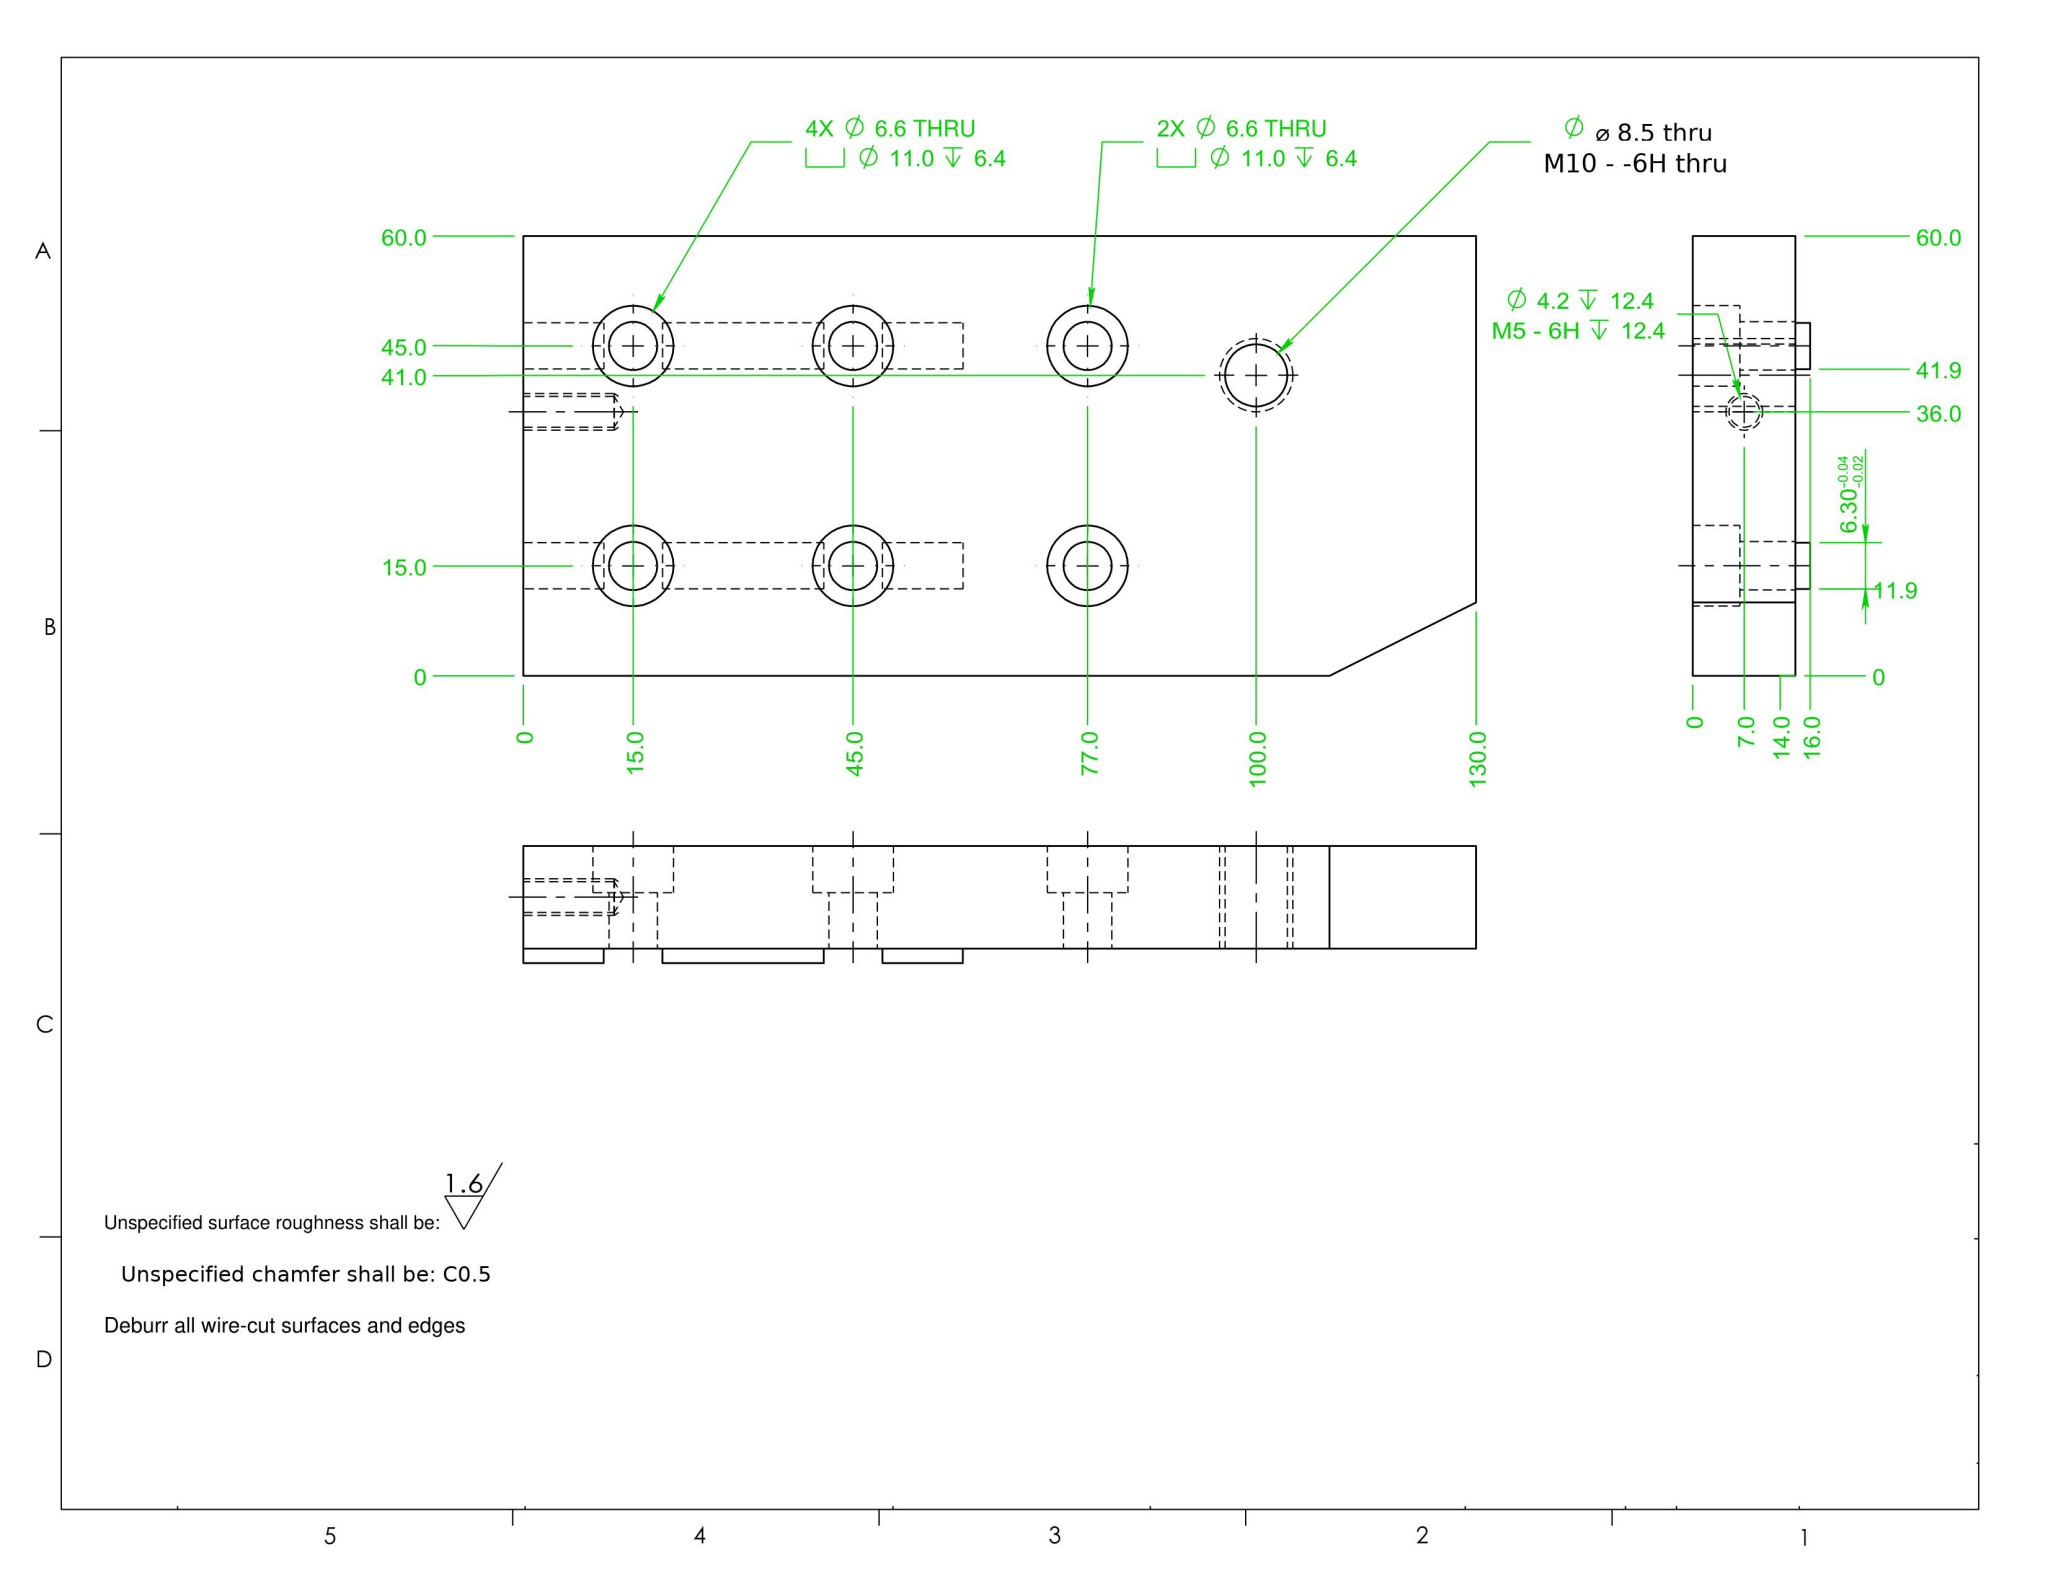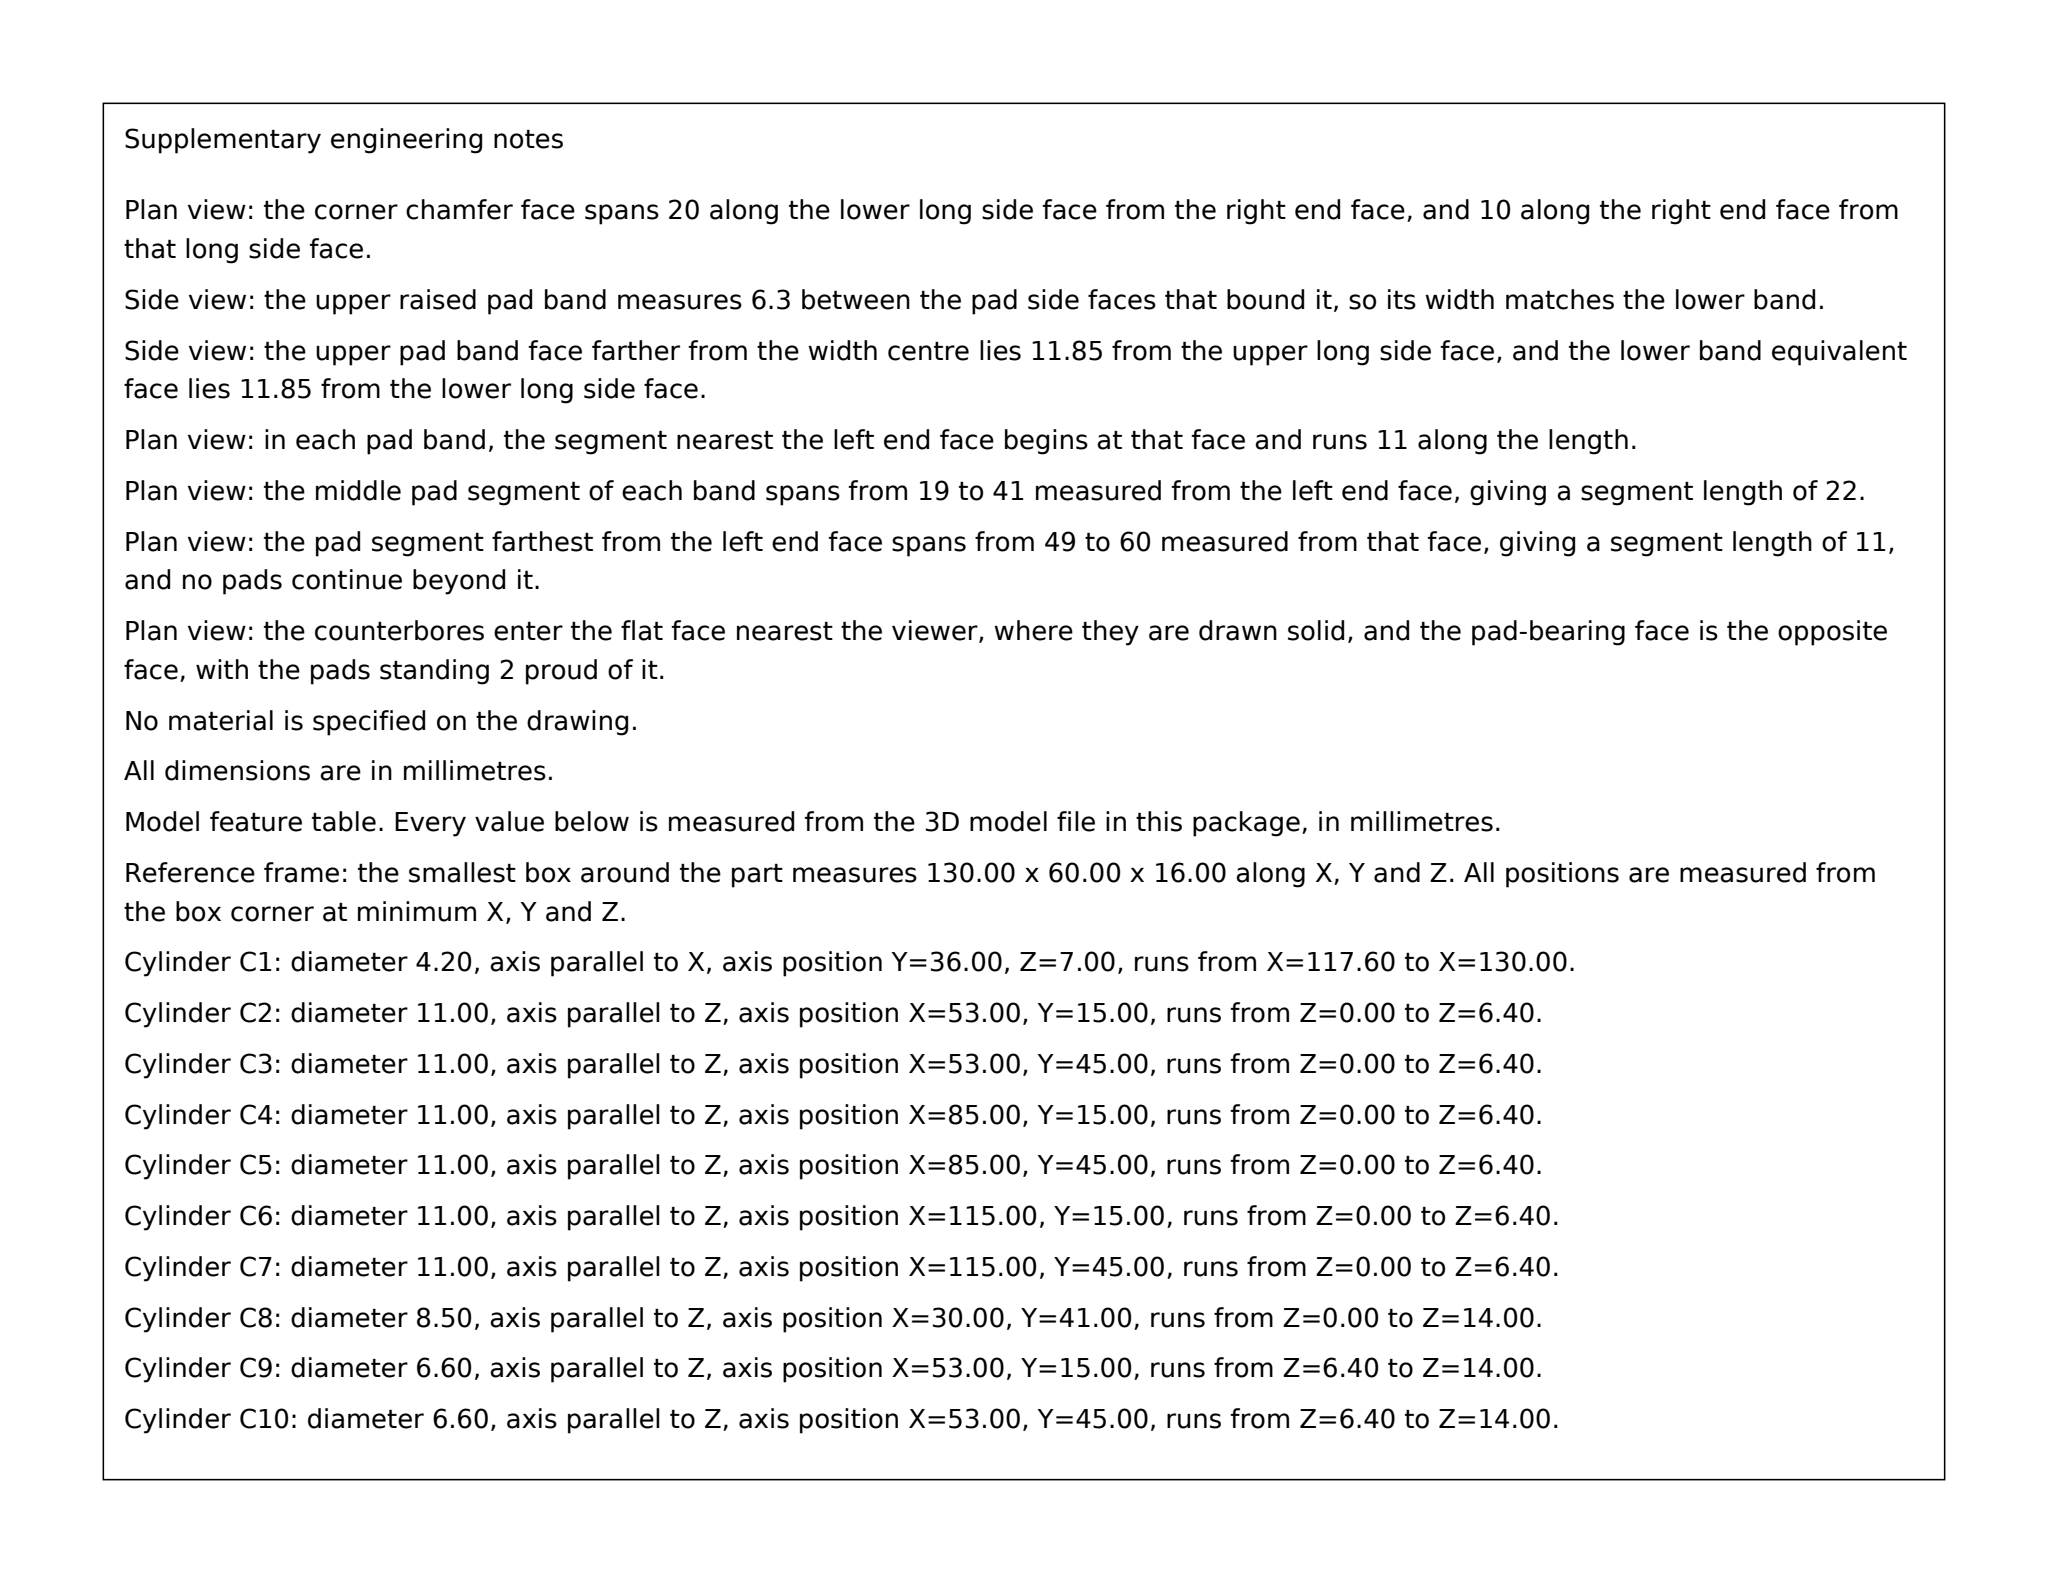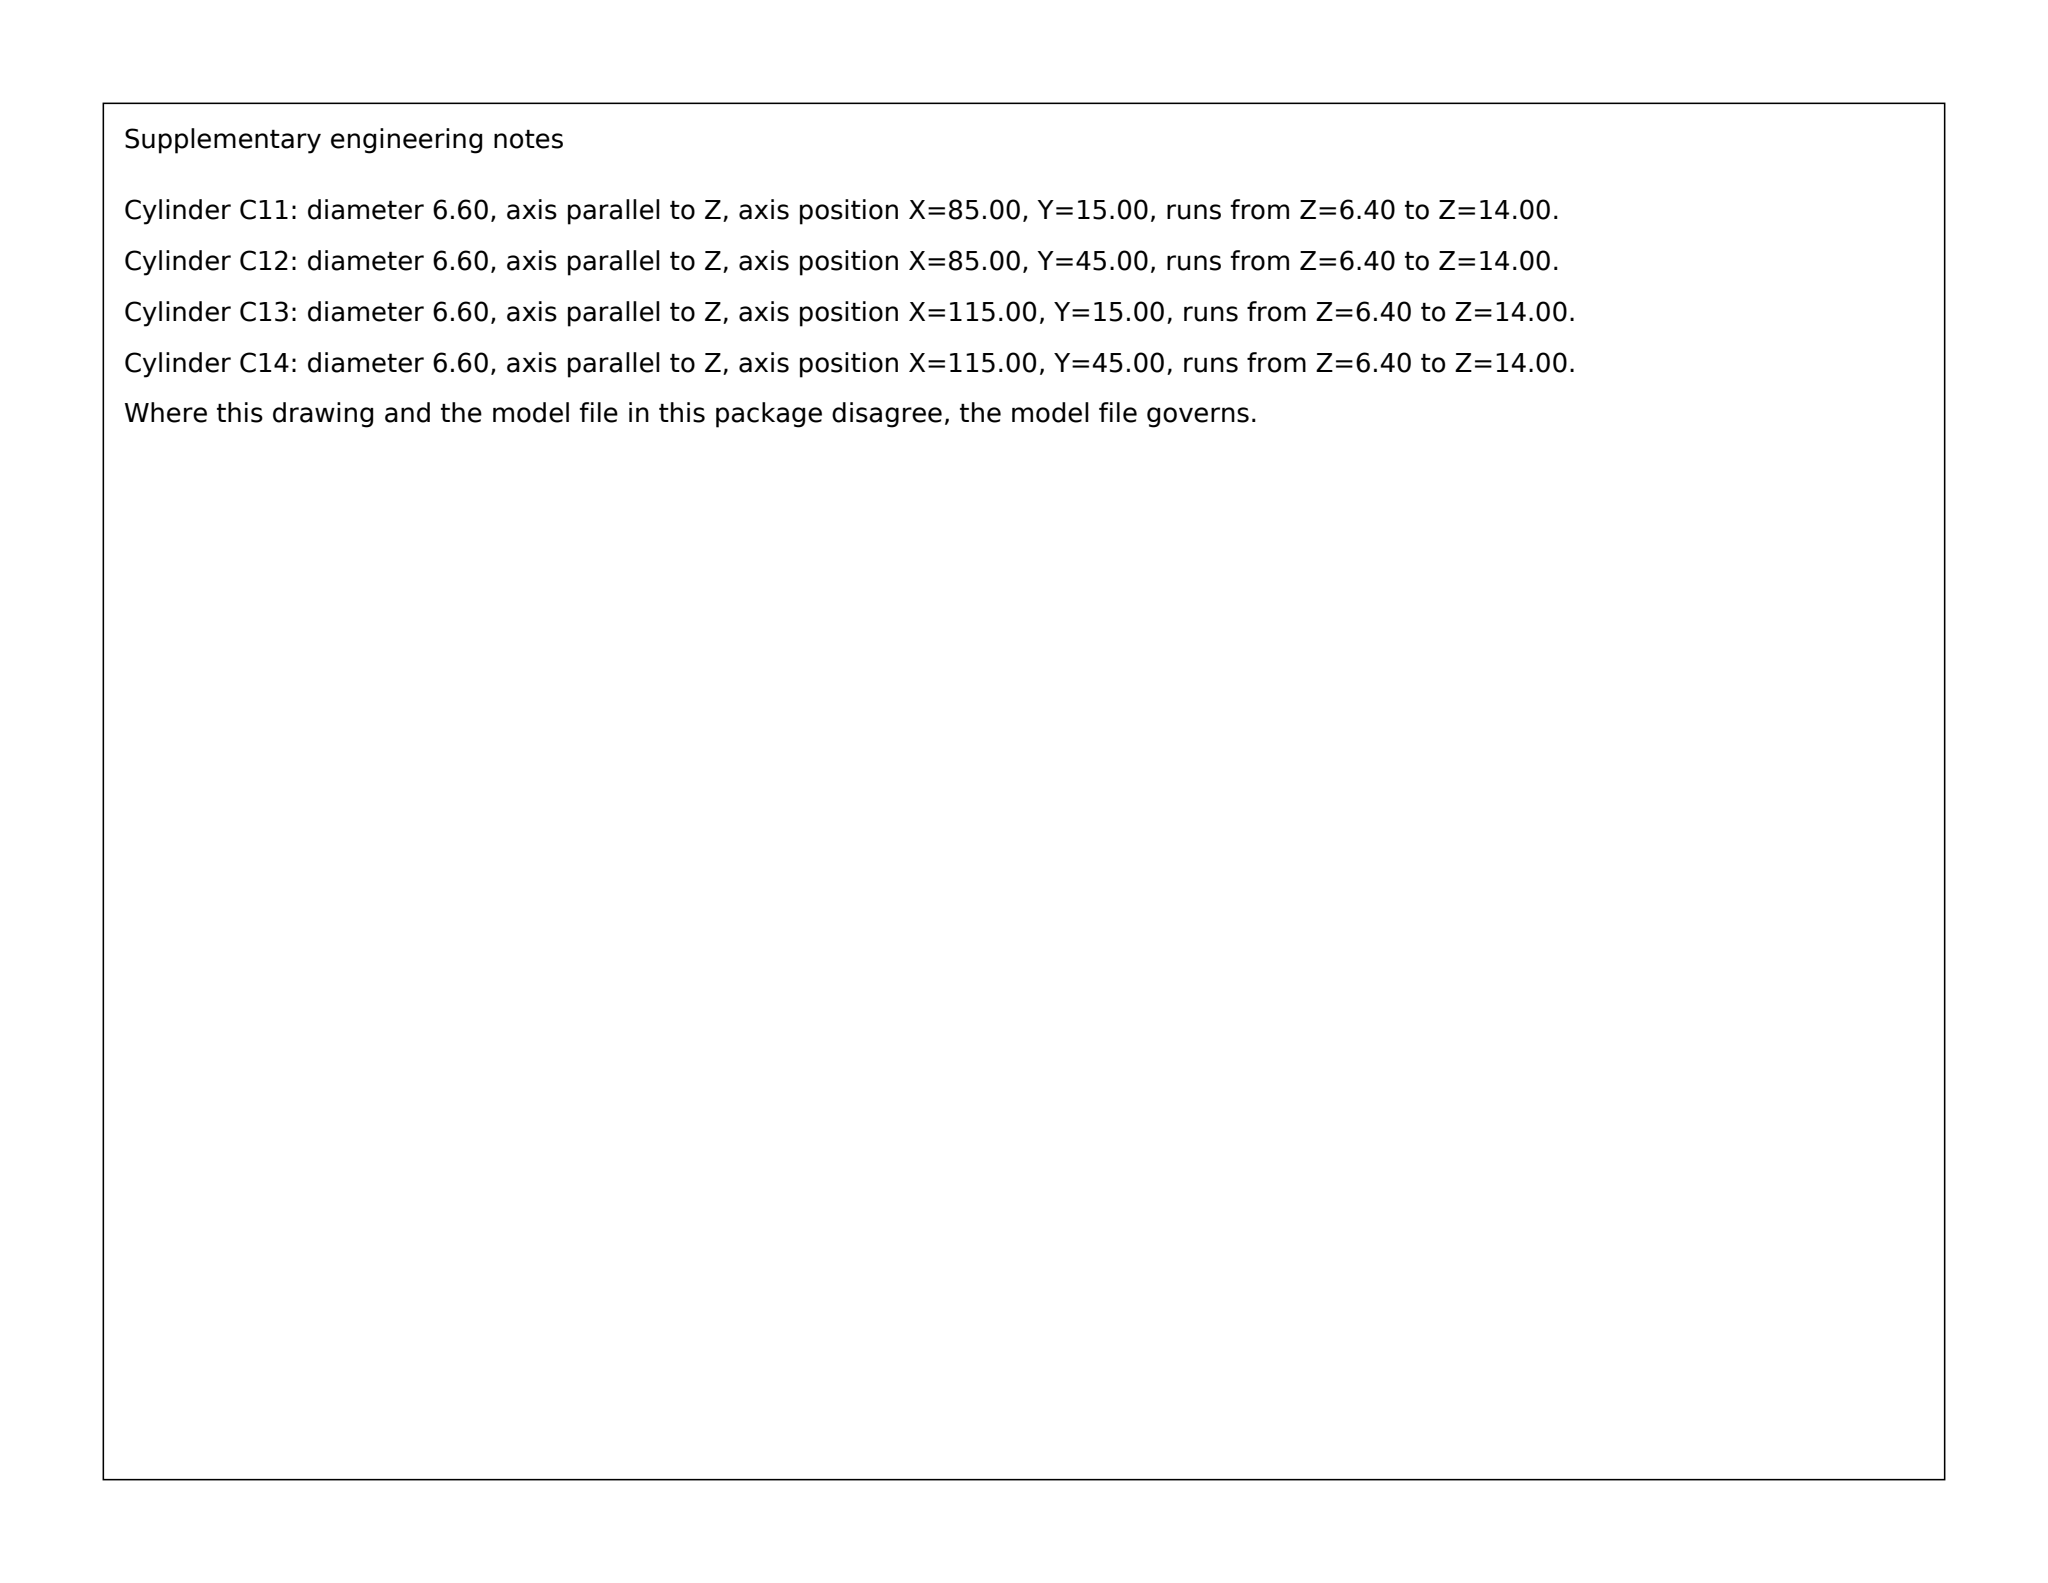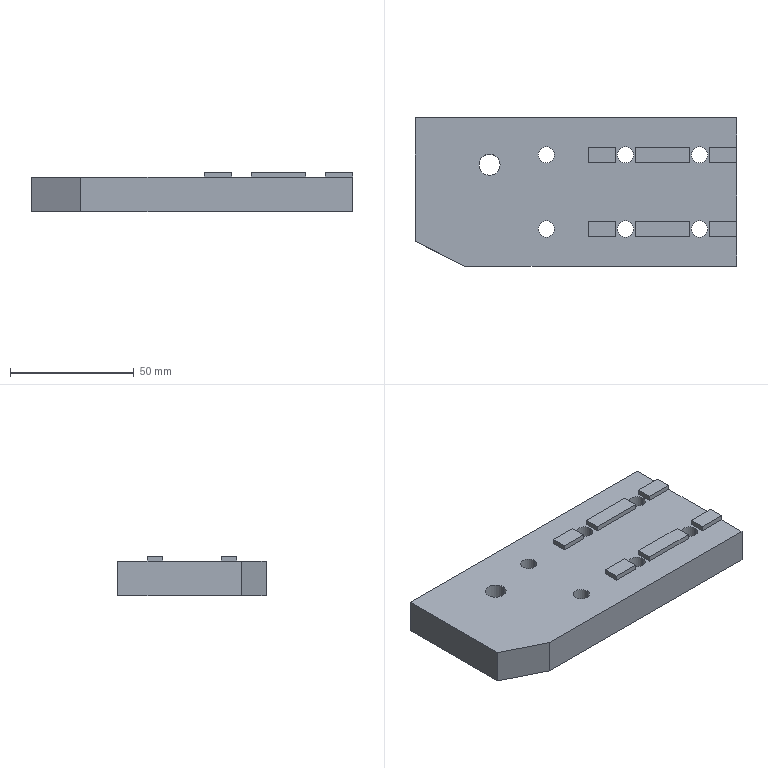Part | SolidWorks | mm | 1 solid | 71 faces | box 130 x 60 x 16 mm | volume 102727 mm3 | plane 41 | cylinder 28 | cone 2 | commonest cylinder face diameters 11 x12 6.6 x12 8.5 x2 4.2 x2
Drawing notes:
PLATE OAL 130 FROM X0 END TO RIGHT END FACE | from the solid: bbox_xyz X = 130.0; axis_planes x = 0.0 and x = 130.0
2X 6.3 WIDE RAILS ON UNDERSIDE RUN 60 FROM X0 END | from the solid: rail faces at x = 70.0 (=130-60) and plate end x = 130.0 (drawing X0); rail width 48.15-41.85 = 6.3, 18.15-11.85 = 6.3
build123d program:
from build123d import *

# Parameters (mm, degrees)
SKETCH1_W                                       = 130
SKETCH1_H                                       = 60
BOSS_EXTRUDE1_DEPTH                             = 14
CHAMFER1_SIZE                                   = 10
CHAMFER1_SIZE2                                  = 20
SKETCH4_W                                       = 60
SKETCH4_H                                       = 6.3
BOSS_EXTRUDE2_DEPTH                             = 2
M6_HEX_SOCKET_HEAD_CAP_SCREW_CBORE1_D           = 6.6
M6_HEX_SOCKET_HEAD_CAP_SCREW_CBORE1_CBORE_D     = 11
M6_HEX_SOCKET_HEAD_CAP_SCREW_CBORE1_CBORE_DEPTH = 6.4
SKETCH8_W                                       = 8
SKETCH8_H                                       = 60
CUT_EXTRUDE1_DEPTH                              = 2
M6_HEX_SOCKET_HEAD_CAP_SCREW_CBORE2_D           = 6.6
M6_HEX_SOCKET_HEAD_CAP_SCREW_CBORE2_CBORE_D     = 11
M6_HEX_SOCKET_HEAD_CAP_SCREW_CBORE2_CBORE_DEPTH = 6.4
M5_TAPPED_HOLE1_D                               = 4.2
M5_TAPPED_HOLE1_DEPTH                           = 12.4
M5_TAPPED_HOLE1_TIP                             = 1.262
M10_TAPPED_HOLE1_D                              = 8.5


with BuildPart() as part:
    # Sketch1 → Boss-Extrude1 (new body)
    with BuildSketch(Plane.XY):
        Rectangle(SKETCH1_W, SKETCH1_H)
    extrude(amount=BOSS_EXTRUDE1_DEPTH)

    # Chamfer1
    chamfer1_edges = [part.edges().sort_by_distance(p)[0] for p in [
        (-65, -30, 7),
    ]]
    chamfer1_side = [part.faces().sort_by_distance(p)[0] for p in [
        (-65, 0, 7),
    ]]
    chamfer(chamfer1_edges, length=CHAMFER1_SIZE, length2=CHAMFER1_SIZE2, reference=chamfer1_side[0])

    # Sketch4 → Boss-Extrude2 (add)
    with BuildSketch(Plane.XY.offset(14)):
        with Locations((35, -15)):
            Rectangle(SKETCH4_W, SKETCH4_H)
        with Locations((35, 15)):
            Rectangle(SKETCH4_W, SKETCH4_H)
    extrude(amount=BOSS_EXTRUDE2_DEPTH)

    # M6 Hex Socket Head Cap Screw CBORE1 (through all)
    with Locations(Plane(origin=(0, 0, 0), x_dir=(-1, 0, 0), z_dir=(0, 0, -1))):
        with Locations((-50, 15), (-20, 15), (-20, -15), (-50, -15)):
            CounterBoreHole(M6_HEX_SOCKET_HEAD_CAP_SCREW_CBORE1_D / 2, M6_HEX_SOCKET_HEAD_CAP_SCREW_CBORE1_CBORE_D / 2, M6_HEX_SOCKET_HEAD_CAP_SCREW_CBORE1_CBORE_DEPTH)

    # Sketch8 → Cut-Extrude1 (cut)
    with BuildSketch(Plane.XY.offset(16)):
        with Locations((20, 0)):
            Rectangle(SKETCH8_W, SKETCH8_H)
        with Locations((50, 0)):
            Rectangle(SKETCH8_W, SKETCH8_H)
    extrude(amount=-CUT_EXTRUDE1_DEPTH, mode=Mode.SUBTRACT)

    # M6 Hex Socket Head Cap Screw CBORE2 (through all)
    with Locations(Plane(origin=(0, 0, 0), x_dir=(-1, 0, 0), z_dir=(0, 0, -1))):
        with Locations((12, 15), (12, -15)):
            CounterBoreHole(M6_HEX_SOCKET_HEAD_CAP_SCREW_CBORE2_D / 2, M6_HEX_SOCKET_HEAD_CAP_SCREW_CBORE2_CBORE_D / 2, M6_HEX_SOCKET_HEAD_CAP_SCREW_CBORE2_CBORE_DEPTH)

    # M5 Tapped Hole1
    with Locations(Plane(origin=(65, 0, 0), x_dir=(0, 0, -1), z_dir=(1, 0, 0))):
        with Locations((-7, 6)):
            Hole(M5_TAPPED_HOLE1_D / 2, depth=M5_TAPPED_HOLE1_DEPTH)
            with Locations((0, 0, -(M5_TAPPED_HOLE1_DEPTH + M5_TAPPED_HOLE1_TIP / 2))):  # 118° drill point
                Cone(0, M5_TAPPED_HOLE1_D / 2, M5_TAPPED_HOLE1_TIP, mode=Mode.SUBTRACT)

    # M10 Tapped Hole1 (through all)
    with Locations(Plane.XY.offset(14)):
        with Locations((-35, 11)):
            Hole(M10_TAPPED_HOLE1_D / 2)


solid = part.part